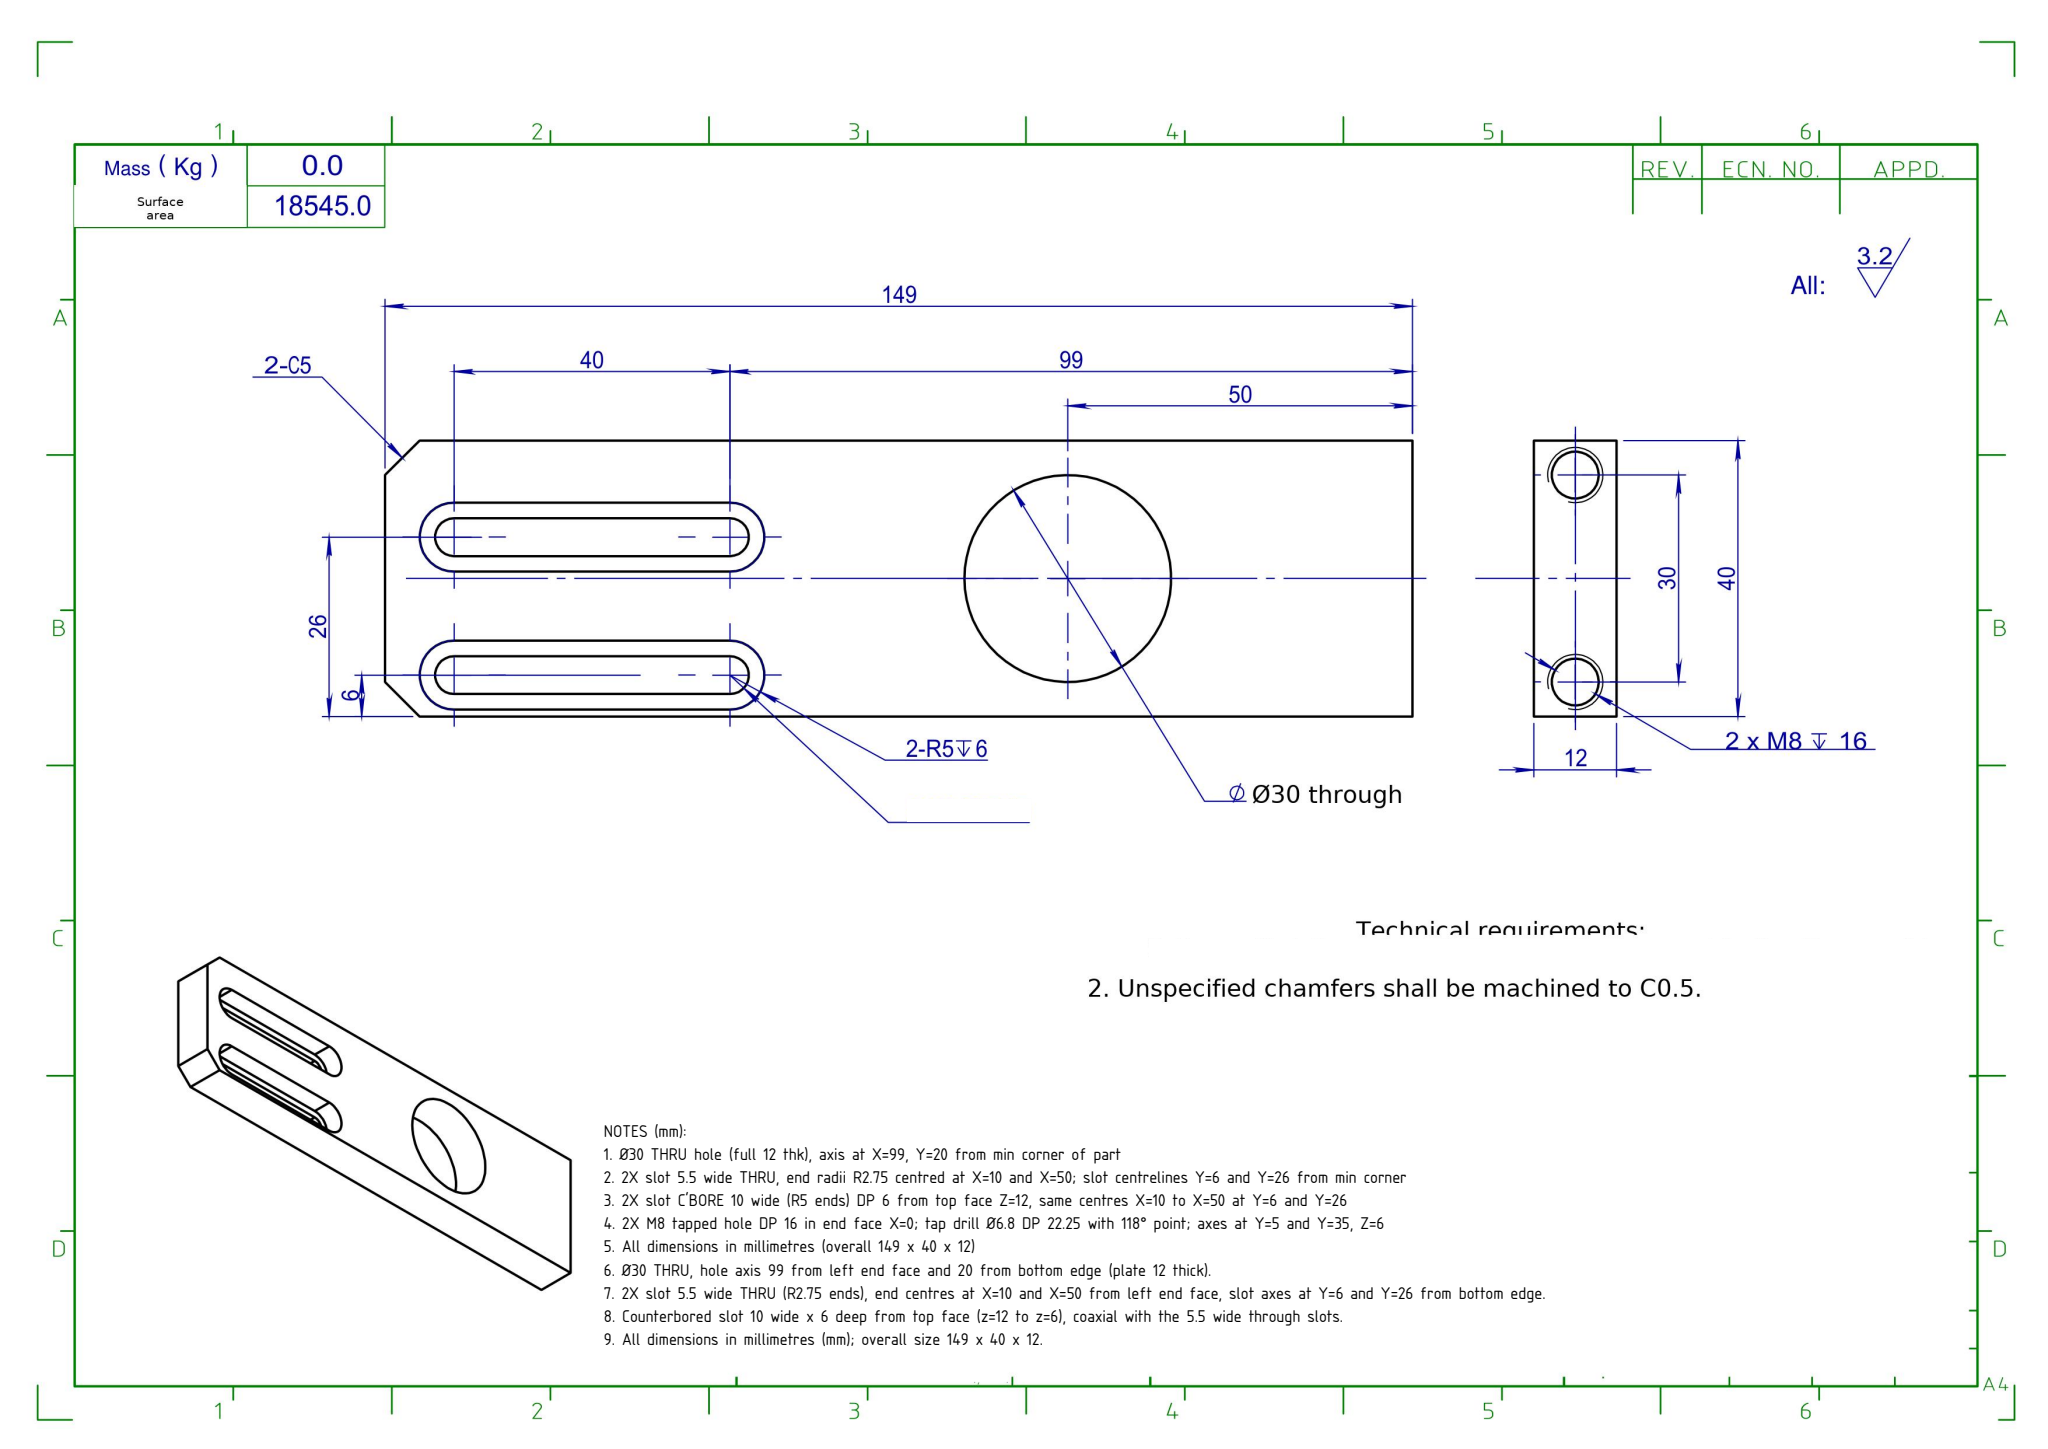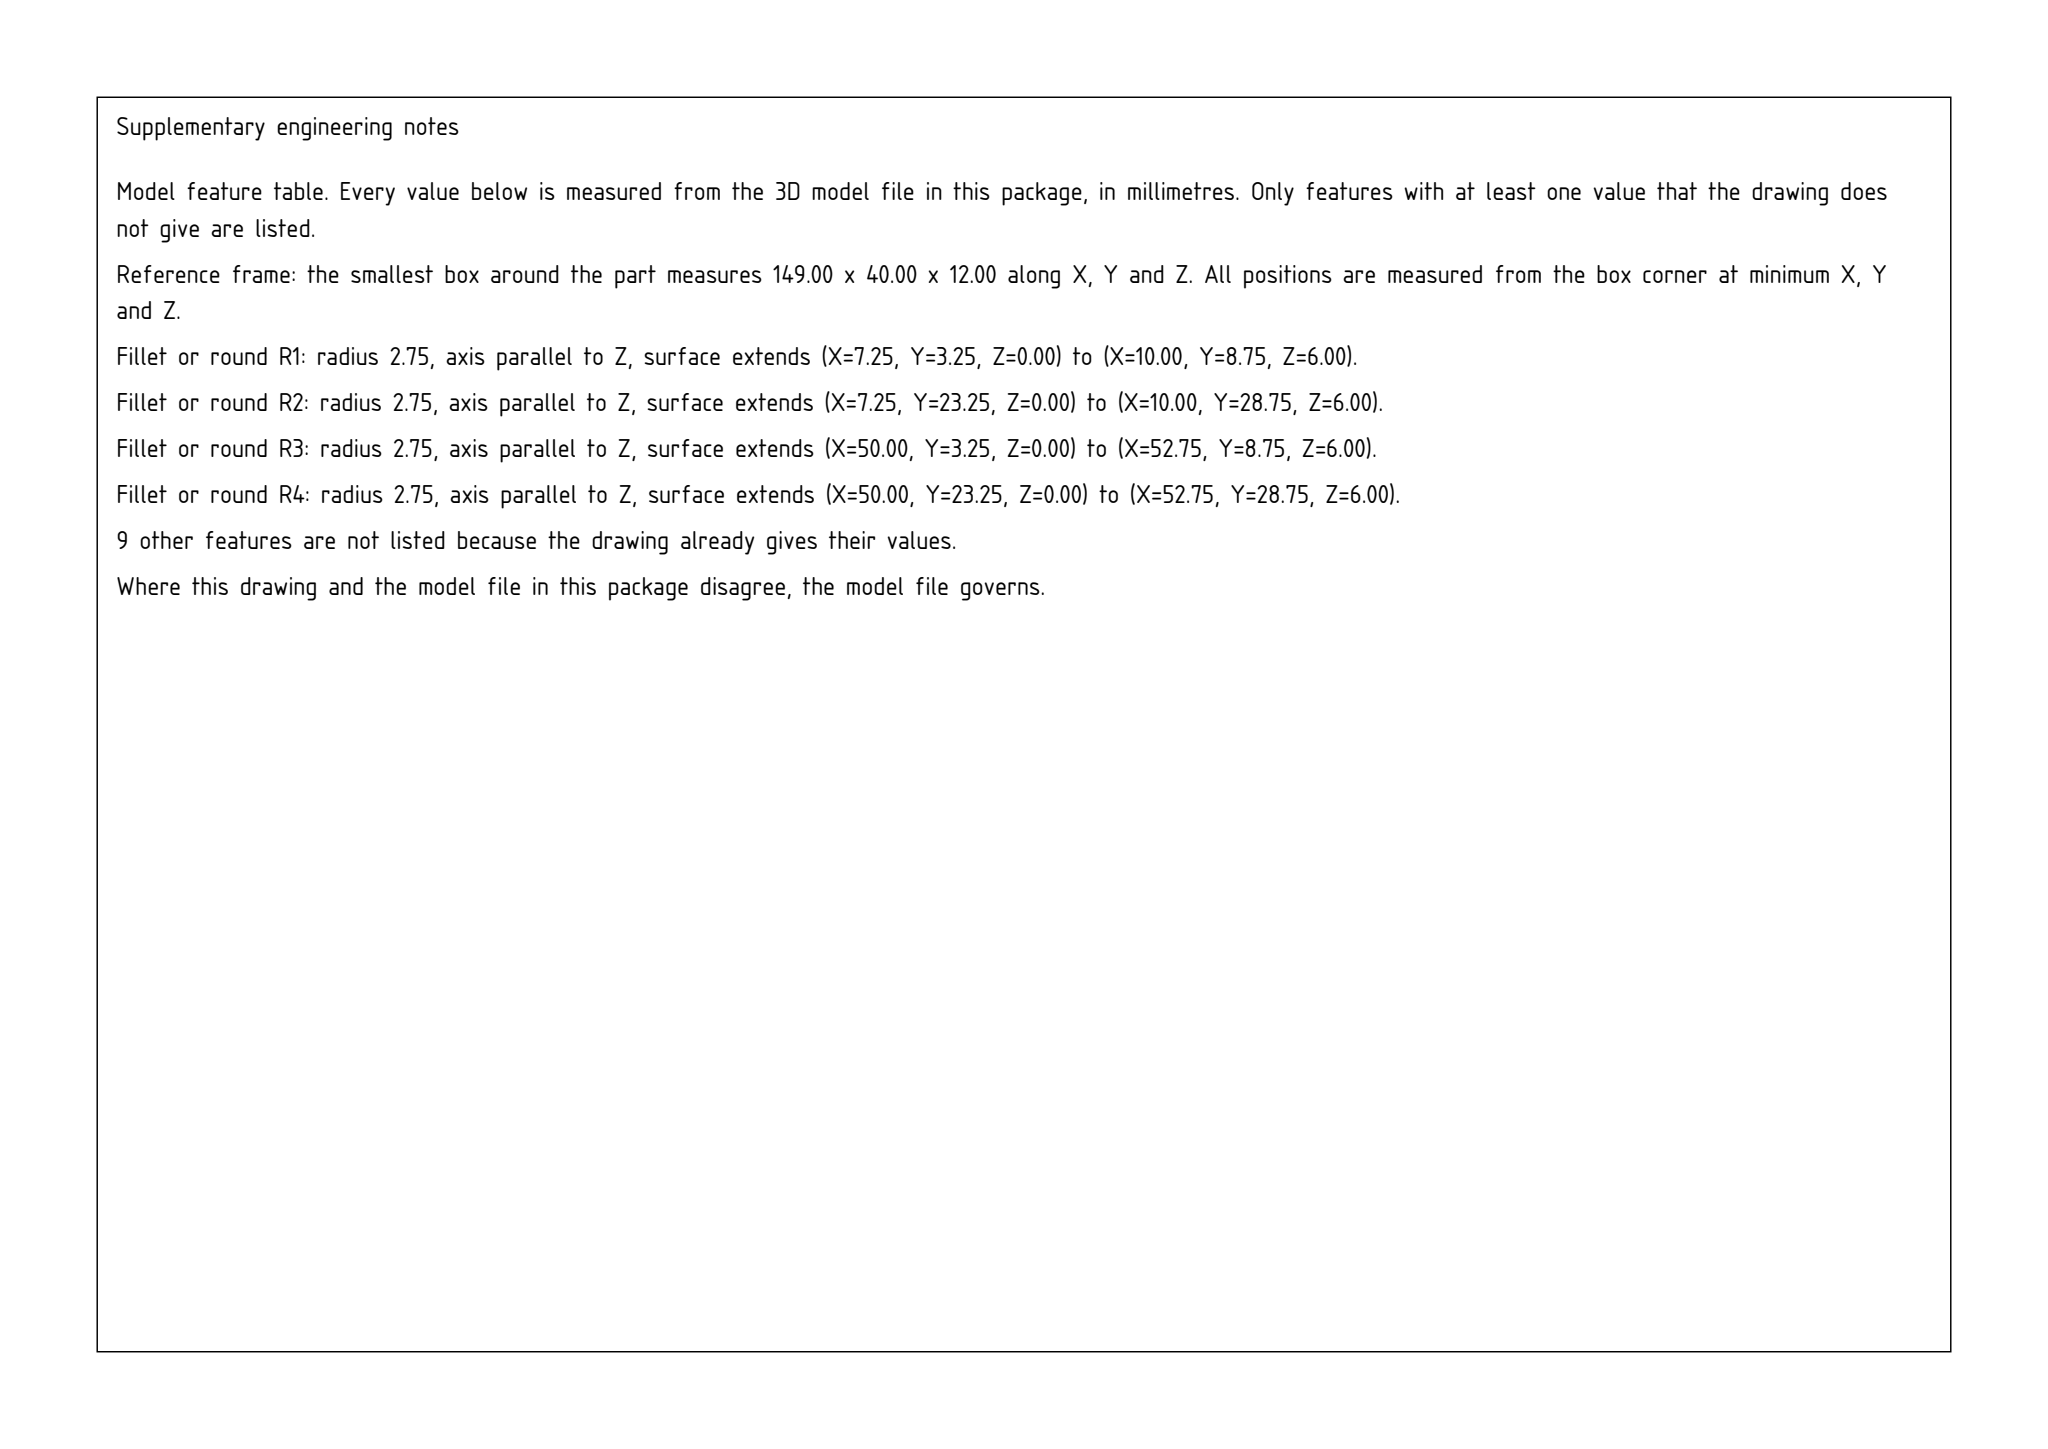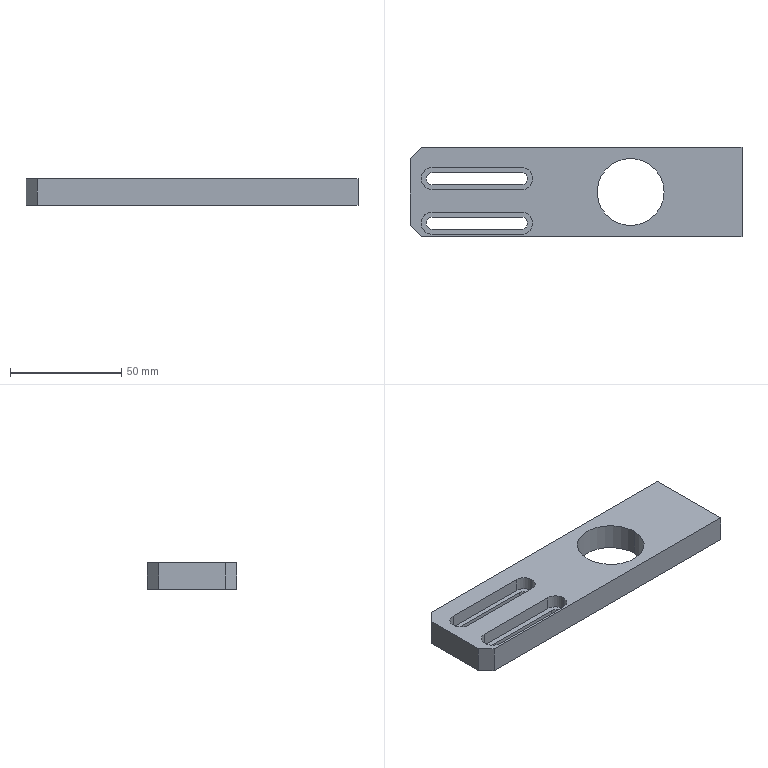Part | SolidWorks | mm | 1 solid | 40 faces | box 149 x 40 x 12 mm | volume 52405 mm3 | cylinder 18 | plane 18 | cone 4 | commonest cylinder face diameters 5.5 x6 10 x6 6.8 x4 30 x2
Drawing notes:
Ø30 THRU hole (full 12 thk), axis at X=99, Y=20 from min corner of part | from the solid: cylinders: [30.0,"z",[99.0,20.0],12.0]
2X slot 5.5 wide THRU, end radii R2.75 centred at X=10 and X=50; slot centrelines Y=6 and Y=26 from min corner | from the solid: cylinders: [5.5,"z",[10.0,6.0]], [5.5,"z",[10.0,26.0]], [5.5,"z",[50.0,6.0]], [5.5,"z",[50.0,26.0]]
2X slot C'BORE 10 wide (R5 ends) DP 6 from top face Z=12, same centres X=10 to X=50 at Y=6 and Y=26 | from the solid: cylinders: [10.0,"z",[10.0,6.0],6.0], [10.0,"z",[50.0,26.0],6.0]; axis_plane z=6.0
2X M8 tapped hole DP 16 in end face X=0; tap drill Ø6.8 DP 22.25 with 118° point; axes at Y=5 and Y=35, Z=6 | from the solid: cylinders: [6.8,"x",[null,5.0,6.0],22.25], [6.8,"x",[null,35.0,6.0],22.25]; cones: [118.0,6.8]
All dimensions in millimetres (overall 149 x 40 x 12) | from the solid: bbox_xyz [149.0,40.0,12.0] in mm
Ø30 THRU, hole axis 99 from left end face and 20 from bottom edge (plate 12 thick). | from the solid: cylinders: [30.0, axis z, pos (99.0, 20.0), length 12.0]
2X slot 5.5 wide THRU (R2.75 ends), end centres at X=10 and X=50 from left end face, slot axes at Y=6 and Y=26 from bottom edge. | from the solid: cylinders: [5.5, axis z, pos (10.0,6.0)/(10.0,26.0)/(50.0,6.0)/(50.0,26.0), length 6.0]
Counterbored slot 10 wide x 6 deep from top face (z=12 to z=6), coaxial with the 5.5 wide through slots. | from the solid: cylinders: [10.0, axis z, pos (10.0,6.0)/(10.0,26.0)/(50.0,6.0)/(50.0,26.0), length 6.0]; axis_planes z=6.0
All dimensions in millimetres (mm); overall size 149 x 40 x 12. | from the solid: bbox_xyz [149.0, 40.0, 12.0] in mm
build123d program:
from build123d import *

# Parameters (mm, degrees)
SKETCH1_W             = 149
SKETCH1_H             = 40
EXTRUDE1_DEPTH        = 12
M8_TAPPED_HOLE1_D     = 6.8
M8_TAPPED_HOLE1_DEPTH = 22.25
M8_TAPPED_HOLE1_TIP   = 2.043
M4_TAPPED_HOLE1_D     = 3.3
SKETCH6_R             = 15
CUT_EXTRUDE1_DEPTH    = 79.066
CHAMFER1_SIZE         = 5
CUT_EXTRUDE2_DEPTH    = 6
CUT_EXTRUDE4_DEPTH    = 78.371


with BuildPart() as part:
    # Sketch1 → Extrude1 (new body)
    with BuildSketch(Plane.XY):
        Rectangle(SKETCH1_W, SKETCH1_H)
    extrude(amount=EXTRUDE1_DEPTH)

    # M8 Tapped Hole1
    with Locations(Plane(origin=(74.5, 0, 0), x_dir=(0, 0, -1), z_dir=(1, 0, 0))):
        with Locations((-6, 15), (-6, -15)):
            Hole(M8_TAPPED_HOLE1_D / 2, depth=M8_TAPPED_HOLE1_DEPTH)
            with Locations((0, 0, -(M8_TAPPED_HOLE1_DEPTH + M8_TAPPED_HOLE1_TIP / 2))):  # 118° drill point
                Cone(0, M8_TAPPED_HOLE1_D / 2, M8_TAPPED_HOLE1_TIP, mode=Mode.SUBTRACT)

    # M4 Tapped Hole1 (through all)
    with Locations(Plane.XY.offset(12)):
        with Locations((-59.5, -14), (-36.5, 6), (-36.5, -14), (-59.5, 6)):
            Hole(M4_TAPPED_HOLE1_D / 2)

    # Sketch6 → Cut-Extrude1 (cut, through all)
    with BuildSketch(Plane(origin=(0, 0, 0), x_dir=(-1, 0, 0), z_dir=(0, 0, -1))):
        with Locations((-24.5, 0)):
            Circle(SKETCH6_R)
    extrude(amount=-CUT_EXTRUDE1_DEPTH, mode=Mode.SUBTRACT)

    # Chamfer1
    chamfer1_edges = [part.edges().sort_by_distance(p)[0] for p in [
        (-74.5, 20, 6),
        (-74.5, -20, 6),
    ]]
    chamfer(chamfer1_edges, length=CHAMFER1_SIZE)

    # Sketch7 → Cut-Extrude2 (cut)
    with BuildSketch(Plane.XY.offset(12)):
        with BuildLine():
            Line((-64.5, 11), (-24.5, 11))
            ThreePointArc((-24.5, 11), (-19.5, 6), (-24.5, 1))
            Line((-24.5, 1), (-64.5, 1))
            ThreePointArc((-64.5, 1), (-69.5, 6), (-64.5, 11))
        make_face()
        with BuildLine():
            Line((-64.5, -9), (-24.5, -9))
            ThreePointArc((-24.5, -9), (-19.5, -14), (-24.5, -19))
            Line((-24.5, -19), (-64.5, -19))
            ThreePointArc((-64.5, -19), (-69.5, -14), (-64.5, -9))
        make_face()
    extrude(amount=-CUT_EXTRUDE2_DEPTH, mode=Mode.SUBTRACT)

    # Sketch8 → Cut-Extrude4 (cut, through all)
    with BuildSketch(Plane.XY.offset(6)):
        with BuildLine():
            Line((-64.5, 3.25), (-24.5, 3.25))
            ThreePointArc((-24.5, 3.25), (-21.75, 6), (-24.5, 8.75))
            Line((-24.5, 8.75), (-64.5, 8.75))
            ThreePointArc((-64.5, 8.75), (-67.25, 6), (-64.5, 3.25))
        make_face()
        with BuildLine():
            Line((-64.5, -16.75), (-24.5, -16.75))
            ThreePointArc((-24.5, -16.75), (-21.75, -14), (-24.5, -11.25))
            Line((-24.5, -11.25), (-64.5, -11.25))
            ThreePointArc((-64.5, -11.25), (-67.25, -14), (-64.5, -16.75))
        make_face()
    extrude(amount=-CUT_EXTRUDE4_DEPTH, mode=Mode.SUBTRACT)


solid = part.part